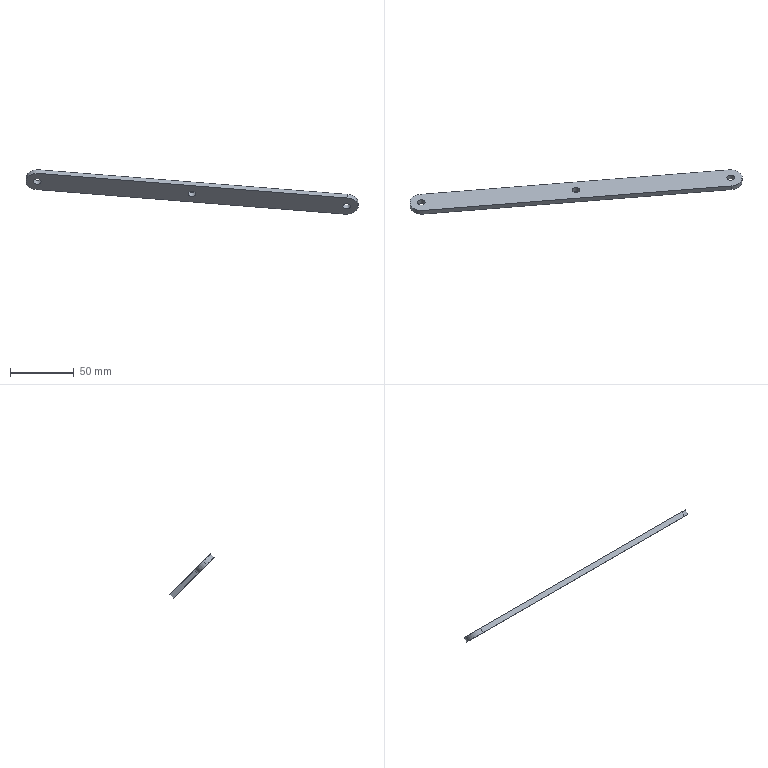Component | SolidWorks | GeneralAssembly-1_TieRod2-1 | 1 solid | 14 faces | box 260.47 x 34.86 x 34.86 mm | volume 18247 mm3 | cylinder 10 | plane 4 | commonest cylinder face diameters 6 x6 18 x4
STEP:
#1=COLOUR_RGB('',0.7922,0.8196,0.9333);
#2=FILL_AREA_STYLE_COLOUR('',#1);
#3=FILL_AREA_STYLE('',(#2));
#4=SURFACE_STYLE_FILL_AREA(#3);
#5=SURFACE_SIDE_STYLE('',(#4));
#6=SURFACE_STYLE_USAGE(.BOTH.,#5);
#7=PRESENTATION_STYLE_ASSIGNMENT((#6));
#8=CARTESIAN_POINT('',(10.928,15.672,-21.042));
#9=VERTEX_POINT('',#8);
#10=CARTESIAN_POINT('',(11.163,15.691,-21.06));
#11=VERTEX_POINT('',#10);
#12=CARTESIAN_POINT('',(11.046,15.682,-21.051));
#13=DIRECTION('',(0.,-0.7071,-0.7071));
#14=DIRECTION('',(0.9937,0.07912,-0.07912));
#15=AXIS2_PLACEMENT_3D('',#12,#13,#14);
#16=CIRCLE('',#15,0.1181);
#17=EDGE_CURVE('',#9,#11,#16,.T.);
#18=ORIENTED_EDGE('',*,*,#17,.F.);
#19=CARTESIAN_POINT('',(10.928,15.561,-21.153));
#20=VERTEX_POINT('',#19);
#21=CARTESIAN_POINT('',(10.928,15.7,-21.014));
#22=DIRECTION('',(0.,-0.7071,-0.7071));
#23=VECTOR('',#22,39.37);
#24=LINE('',#21,#23);
#25=EDGE_CURVE('',#9,#20,#24,.T.);
#26=ORIENTED_EDGE('',*,*,#25,.T.);
#27=CARTESIAN_POINT('',(11.163,15.58,-21.172));
#28=VERTEX_POINT('',#27);
#29=CARTESIAN_POINT('',(11.046,15.57,-21.162));
#30=DIRECTION('',(0.,-0.7071,-0.7071));
#31=DIRECTION('',(0.9937,0.07912,-0.07912));
#32=AXIS2_PLACEMENT_3D('',#29,#30,#31);
#33=CIRCLE('',#32,0.1181);
#34=EDGE_CURVE('',#20,#28,#33,.T.);
#35=ORIENTED_EDGE('',*,*,#34,.T.);
#36=CARTESIAN_POINT('',(11.163,15.719,-21.032));
#37=DIRECTION('',(0.,-0.7071,-0.7071));
#38=VECTOR('',#37,39.37);
#39=LINE('',#36,#38);
#40=EDGE_CURVE('',#11,#28,#39,.T.);
#41=ORIENTED_EDGE('',*,*,#40,.F.);
#42=EDGE_LOOP('',(#18,#26,#35,#41));
#43=FACE_OUTER_BOUND('',#42,.T.);
#44=CARTESIAN_POINT('',(11.046,15.709,-21.023));
#45=DIRECTION('',(0.,-0.7071,-0.7071));
#46=DIRECTION('',(0.9937,0.07912,-0.07912));
#47=AXIS2_PLACEMENT_3D('',#44,#45,#46);
#48=CYLINDRICAL_SURFACE('',#47,0.1181);
#49=ADVANCED_FACE('',(#43),#48,.F.);
#50=CARTESIAN_POINT('',(6.155,15.292,-20.662));
#51=VERTEX_POINT('',#50);
#52=CARTESIAN_POINT('',(6.39,15.311,-20.68));
#53=VERTEX_POINT('',#52);
#54=CARTESIAN_POINT('',(6.273,15.302,-20.671));
#55=DIRECTION('',(0.,-0.7071,-0.7071));
#56=DIRECTION('',(0.9937,0.07912,-0.07912));
#57=AXIS2_PLACEMENT_3D('',#54,#55,#56);
#58=CIRCLE('',#57,0.1181);
#59=EDGE_CURVE('',#51,#53,#58,.T.);
#60=ORIENTED_EDGE('',*,*,#59,.F.);
#61=CARTESIAN_POINT('',(6.155,15.181,-20.773));
#62=VERTEX_POINT('',#61);
#63=CARTESIAN_POINT('',(6.155,15.32,-20.634));
#64=DIRECTION('',(0.,-0.7071,-0.7071));
#65=VECTOR('',#64,39.37);
#66=LINE('',#63,#65);
#67=EDGE_CURVE('',#51,#62,#66,.T.);
#68=ORIENTED_EDGE('',*,*,#67,.T.);
#69=CARTESIAN_POINT('',(6.39,15.2,-20.792));
#70=VERTEX_POINT('',#69);
#71=CARTESIAN_POINT('',(6.273,15.19,-20.782));
#72=DIRECTION('',(0.,-0.7071,-0.7071));
#73=DIRECTION('',(0.9937,0.07912,-0.07912));
#74=AXIS2_PLACEMENT_3D('',#71,#72,#73);
#75=CIRCLE('',#74,0.1181);
#76=EDGE_CURVE('',#62,#70,#75,.T.);
#77=ORIENTED_EDGE('',*,*,#76,.T.);
#78=CARTESIAN_POINT('',(6.39,15.339,-20.652));
#79=DIRECTION('',(0.,-0.7071,-0.7071));
#80=VECTOR('',#79,39.37);
#81=LINE('',#78,#80);
#82=EDGE_CURVE('',#53,#70,#81,.T.);
#83=ORIENTED_EDGE('',*,*,#82,.F.);
#84=EDGE_LOOP('',(#60,#68,#77,#83));
#85=FACE_OUTER_BOUND('',#84,.T.);
#86=CARTESIAN_POINT('',(6.273,15.329,-20.643));
#87=DIRECTION('',(0.,-0.7071,-0.7071));
#88=DIRECTION('',(0.9937,0.07912,-0.07912));
#89=AXIS2_PLACEMENT_3D('',#86,#87,#88);
#90=CYLINDRICAL_SURFACE('',#89,0.1181);
#91=ADVANCED_FACE('',(#85),#90,.F.);
#92=CARTESIAN_POINT('',(1.382,14.912,-20.282));
#93=VERTEX_POINT('',#92);
#94=CARTESIAN_POINT('',(1.617,14.931,-20.3));
#95=VERTEX_POINT('',#94);
#96=CARTESIAN_POINT('',(1.5,14.921,-20.291));
#97=DIRECTION('',(0.,-0.7071,-0.7071));
#98=DIRECTION('',(0.9937,0.07912,-0.07912));
#99=AXIS2_PLACEMENT_3D('',#96,#97,#98);
#100=CIRCLE('',#99,0.1181);
#101=EDGE_CURVE('',#93,#95,#100,.T.);
#102=ORIENTED_EDGE('',*,*,#101,.F.);
#103=CARTESIAN_POINT('',(1.382,14.801,-20.393));
#104=VERTEX_POINT('',#103);
#105=CARTESIAN_POINT('',(1.382,14.94,-20.254));
#106=DIRECTION('',(0.,-0.7071,-0.7071));
#107=VECTOR('',#106,39.37);
#108=LINE('',#105,#107);
#109=EDGE_CURVE('',#93,#104,#108,.T.);
#110=ORIENTED_EDGE('',*,*,#109,.T.);
#111=CARTESIAN_POINT('',(1.617,14.819,-20.412));
#112=VERTEX_POINT('',#111);
#113=CARTESIAN_POINT('',(1.5,14.81,-20.402));
#114=DIRECTION('',(0.,-0.7071,-0.7071));
#115=DIRECTION('',(0.9937,0.07912,-0.07912));
#116=AXIS2_PLACEMENT_3D('',#113,#114,#115);
#117=CIRCLE('',#116,0.1181);
#118=EDGE_CURVE('',#104,#112,#117,.T.);
#119=ORIENTED_EDGE('',*,*,#118,.T.);
#120=CARTESIAN_POINT('',(1.617,14.959,-20.272));
#121=DIRECTION('',(0.,-0.7071,-0.7071));
#122=VECTOR('',#121,39.37);
#123=LINE('',#120,#122);
#124=EDGE_CURVE('',#95,#112,#123,.T.);
#125=ORIENTED_EDGE('',*,*,#124,.F.);
#126=EDGE_LOOP('',(#102,#110,#119,#125));
#127=FACE_OUTER_BOUND('',#126,.T.);
#128=CARTESIAN_POINT('',(1.5,14.949,-20.263));
#129=DIRECTION('',(0.,-0.7071,-0.7071));
#130=DIRECTION('',(0.9937,0.07912,-0.07912));
#131=AXIS2_PLACEMENT_3D('',#128,#129,#130);
#132=CYLINDRICAL_SURFACE('',#131,0.1181);
#133=ADVANCED_FACE('',(#127),#132,.F.);
#134=CARTESIAN_POINT('',(1.46,15.17,-20.54));
#135=VERTEX_POINT('',#134);
#136=CARTESIAN_POINT('',(11.006,15.931,-21.3));
#137=VERTEX_POINT('',#136);
#138=CARTESIAN_POINT('',(1.108,15.142,-20.512));
#139=DIRECTION('',(0.9937,0.07912,-0.07912));
#140=VECTOR('',#139,39.37);
#141=LINE('',#138,#140);
#142=EDGE_CURVE('',#135,#137,#141,.T.);
#143=ORIENTED_EDGE('',*,*,#142,.T.);
#144=CARTESIAN_POINT('',(11.006,15.819,-21.411));
#145=VERTEX_POINT('',#144);
#146=CARTESIAN_POINT('',(11.006,15.819,-21.411));
#147=DIRECTION('',(0.,-0.7071,-0.7071));
#148=VECTOR('',#147,39.37);
#149=LINE('',#146,#148);
#150=EDGE_CURVE('',#137,#145,#149,.T.);
#151=ORIENTED_EDGE('',*,*,#150,.T.);
#152=CARTESIAN_POINT('',(1.46,15.059,-20.651));
#153=VERTEX_POINT('',#152);
#154=CARTESIAN_POINT('',(1.108,15.031,-20.623));
#155=DIRECTION('',(0.9937,0.07912,-0.07912));
#156=VECTOR('',#155,39.37);
#157=LINE('',#154,#156);
#158=EDGE_CURVE('',#153,#145,#157,.T.);
#159=ORIENTED_EDGE('',*,*,#158,.F.);
#160=CARTESIAN_POINT('',(1.46,15.059,-20.651));
#161=DIRECTION('',(-0.,0.7071,0.7071));
#162=VECTOR('',#161,39.37);
#163=LINE('',#160,#162);
#164=EDGE_CURVE('',#153,#135,#163,.T.);
#165=ORIENTED_EDGE('',*,*,#164,.T.);
#166=EDGE_LOOP('',(#143,#151,#159,#165));
#167=FACE_OUTER_BOUND('',#166,.T.);
#168=CARTESIAN_POINT('',(1.108,15.031,-20.623));
#169=DIRECTION('',(0.1119,-0.7027,0.7027));
#170=DIRECTION('',(0.,-0.7071,-0.7071));
#171=AXIS2_PLACEMENT_3D('',#168,#169,#170);
#172=PLANE('',#171);
#173=ADVANCED_FACE('',(#167),#172,.F.);
#174=CARTESIAN_POINT('',(11.085,15.321,-20.913));
#175=VERTEX_POINT('',#174);
#176=CARTESIAN_POINT('',(1.539,14.561,-20.153));
#177=VERTEX_POINT('',#176);
#178=CARTESIAN_POINT('',(1.187,14.533,-20.125));
#179=DIRECTION('',(-0.9937,-0.07912,0.07912));
#180=VECTOR('',#179,39.37);
#181=LINE('',#178,#180);
#182=EDGE_CURVE('',#175,#177,#181,.T.);
#183=ORIENTED_EDGE('',*,*,#182,.F.);
#184=CARTESIAN_POINT('',(11.085,15.433,-20.802));
#185=VERTEX_POINT('',#184);
#186=CARTESIAN_POINT('',(11.085,15.321,-20.913));
#187=DIRECTION('',(-0.,0.7071,0.7071));
#188=VECTOR('',#187,39.37);
#189=LINE('',#186,#188);
#190=EDGE_CURVE('',#175,#185,#189,.T.);
#191=ORIENTED_EDGE('',*,*,#190,.T.);
#192=CARTESIAN_POINT('',(1.539,14.673,-20.042));
#193=VERTEX_POINT('',#192);
#194=CARTESIAN_POINT('',(1.187,14.644,-20.014));
#195=DIRECTION('',(-0.9937,-0.07912,0.07912));
#196=VECTOR('',#195,39.37);
#197=LINE('',#194,#196);
#198=EDGE_CURVE('',#185,#193,#197,.T.);
#199=ORIENTED_EDGE('',*,*,#198,.T.);
#200=CARTESIAN_POINT('',(1.539,14.561,-20.153));
#201=DIRECTION('',(0.,-0.7071,-0.7071));
#202=VECTOR('',#201,39.37);
#203=LINE('',#200,#202);
#204=EDGE_CURVE('',#193,#177,#203,.T.);
#205=ORIENTED_EDGE('',*,*,#204,.T.);
#206=EDGE_LOOP('',(#183,#191,#199,#205));
#207=FACE_OUTER_BOUND('',#206,.T.);
#208=CARTESIAN_POINT('',(1.187,14.533,-20.125));
#209=DIRECTION('',(-0.1119,0.7027,-0.7027));
#210=DIRECTION('',(-0.,0.7071,0.7071));
#211=AXIS2_PLACEMENT_3D('',#208,#209,#210);
#212=PLANE('',#211);
#213=ADVANCED_FACE('',(#207),#212,.F.);
#214=CARTESIAN_POINT('',(11.046,15.57,-21.162));
#215=DIRECTION('',(0.,-0.7071,-0.7071));
#216=DIRECTION('',(0.9937,0.07912,-0.07912));
#217=AXIS2_PLACEMENT_3D('',#214,#215,#216);
#218=CIRCLE('',#217,0.1181);
#219=EDGE_CURVE('',#28,#20,#218,.T.);
#220=ORIENTED_EDGE('',*,*,#219,.F.);
#221=ORIENTED_EDGE('',*,*,#34,.F.);
#222=EDGE_LOOP('',(#220,#221));
#223=FACE_BOUND('',#222,.T.);
#224=CARTESIAN_POINT('',(6.273,15.19,-20.782));
#225=DIRECTION('',(0.,-0.7071,-0.7071));
#226=DIRECTION('',(0.9937,0.07912,-0.07912));
#227=AXIS2_PLACEMENT_3D('',#224,#225,#226);
#228=CIRCLE('',#227,0.1181);
#229=EDGE_CURVE('',#70,#62,#228,.T.);
#230=ORIENTED_EDGE('',*,*,#229,.F.);
#231=ORIENTED_EDGE('',*,*,#76,.F.);
#232=EDGE_LOOP('',(#230,#231));
#233=FACE_BOUND('',#232,.T.);
#234=CARTESIAN_POINT('',(1.5,14.81,-20.402));
#235=DIRECTION('',(0.,-0.7071,-0.7071));
#236=DIRECTION('',(0.9937,0.07912,-0.07912));
#237=AXIS2_PLACEMENT_3D('',#234,#235,#236);
#238=CIRCLE('',#237,0.1181);
#239=EDGE_CURVE('',#112,#104,#238,.T.);
#240=ORIENTED_EDGE('',*,*,#239,.F.);
#241=ORIENTED_EDGE('',*,*,#118,.F.);
#242=EDGE_LOOP('',(#240,#241));
#243=FACE_BOUND('',#242,.T.);
#244=ORIENTED_EDGE('',*,*,#158,.T.);
#245=CARTESIAN_POINT('',(11.398,15.598,-21.19));
#246=VERTEX_POINT('',#245);
#247=CARTESIAN_POINT('',(11.046,15.57,-21.162));
#248=DIRECTION('',(0.,-0.7071,-0.7071));
#249=DIRECTION('',(0.9937,0.07912,-0.07912));
#250=AXIS2_PLACEMENT_3D('',#247,#248,#249);
#251=CIRCLE('',#250,0.3543);
#252=EDGE_CURVE('',#145,#246,#251,.T.);
#253=ORIENTED_EDGE('',*,*,#252,.T.);
#254=CARTESIAN_POINT('',(11.046,15.57,-21.162));
#255=DIRECTION('',(0.,-0.7071,-0.7071));
#256=DIRECTION('',(0.9937,0.07912,-0.07912));
#257=AXIS2_PLACEMENT_3D('',#254,#255,#256);
#258=CIRCLE('',#257,0.3543);
#259=EDGE_CURVE('',#246,#175,#258,.T.);
#260=ORIENTED_EDGE('',*,*,#259,.T.);
#261=ORIENTED_EDGE('',*,*,#182,.T.);
#262=CARTESIAN_POINT('',(1.148,14.782,-20.374));
#263=VERTEX_POINT('',#262);
#264=CARTESIAN_POINT('',(1.5,14.81,-20.402));
#265=DIRECTION('',(0.,-0.7071,-0.7071));
#266=DIRECTION('',(0.9937,0.07912,-0.07912));
#267=AXIS2_PLACEMENT_3D('',#264,#265,#266);
#268=CIRCLE('',#267,0.3543);
#269=EDGE_CURVE('',#177,#263,#268,.T.);
#270=ORIENTED_EDGE('',*,*,#269,.T.);
#271=CARTESIAN_POINT('',(1.5,14.81,-20.402));
#272=DIRECTION('',(0.,-0.7071,-0.7071));
#273=DIRECTION('',(0.9937,0.07912,-0.07912));
#274=AXIS2_PLACEMENT_3D('',#271,#272,#273);
#275=CIRCLE('',#274,0.3543);
#276=EDGE_CURVE('',#263,#153,#275,.T.);
#277=ORIENTED_EDGE('',*,*,#276,.T.);
#278=EDGE_LOOP('',(#244,#253,#260,#261,#270,#277));
#279=FACE_OUTER_BOUND('',#278,.T.);
#280=CARTESIAN_POINT('',(3.616,15.166,-20.758));
#281=DIRECTION('',(0.,-0.7071,-0.7071));
#282=DIRECTION('',(0.9937,0.07912,-0.07912));
#283=AXIS2_PLACEMENT_3D('',#280,#281,#282);
#284=PLANE('',#283);
#285=ADVANCED_FACE('',(#223,#233,#243,#279),#284,.T.);
#286=CARTESIAN_POINT('',(11.046,15.682,-21.051));
#287=DIRECTION('',(0.,-0.7071,-0.7071));
#288=DIRECTION('',(0.9937,0.07912,-0.07912));
#289=AXIS2_PLACEMENT_3D('',#286,#287,#288);
#290=CIRCLE('',#289,0.1181);
#291=EDGE_CURVE('',#11,#9,#290,.T.);
#292=ORIENTED_EDGE('',*,*,#291,.T.);
#293=ORIENTED_EDGE('',*,*,#17,.T.);
#294=EDGE_LOOP('',(#292,#293));
#295=FACE_BOUND('',#294,.T.);
#296=CARTESIAN_POINT('',(6.273,15.302,-20.671));
#297=DIRECTION('',(0.,-0.7071,-0.7071));
#298=DIRECTION('',(0.9937,0.07912,-0.07912));
#299=AXIS2_PLACEMENT_3D('',#296,#297,#298);
#300=CIRCLE('',#299,0.1181);
#301=EDGE_CURVE('',#53,#51,#300,.T.);
#302=ORIENTED_EDGE('',*,*,#301,.T.);
#303=ORIENTED_EDGE('',*,*,#59,.T.);
#304=EDGE_LOOP('',(#302,#303));
#305=FACE_BOUND('',#304,.T.);
#306=CARTESIAN_POINT('',(1.5,14.921,-20.291));
#307=DIRECTION('',(0.,-0.7071,-0.7071));
#308=DIRECTION('',(0.9937,0.07912,-0.07912));
#309=AXIS2_PLACEMENT_3D('',#306,#307,#308);
#310=CIRCLE('',#309,0.1181);
#311=EDGE_CURVE('',#95,#93,#310,.T.);
#312=ORIENTED_EDGE('',*,*,#311,.T.);
#313=ORIENTED_EDGE('',*,*,#101,.T.);
#314=EDGE_LOOP('',(#312,#313));
#315=FACE_BOUND('',#314,.T.);
#316=CARTESIAN_POINT('',(11.398,15.71,-21.079));
#317=VERTEX_POINT('',#316);
#318=CARTESIAN_POINT('',(11.046,15.682,-21.051));
#319=DIRECTION('',(-0.,0.7071,0.7071));
#320=DIRECTION('',(0.9937,0.07912,-0.07912));
#321=AXIS2_PLACEMENT_3D('',#318,#319,#320);
#322=CIRCLE('',#321,0.3543);
#323=EDGE_CURVE('',#185,#317,#322,.T.);
#324=ORIENTED_EDGE('',*,*,#323,.T.);
#325=CARTESIAN_POINT('',(11.046,15.682,-21.051));
#326=DIRECTION('',(-0.,0.7071,0.7071));
#327=DIRECTION('',(0.9937,0.07912,-0.07912));
#328=AXIS2_PLACEMENT_3D('',#325,#326,#327);
#329=CIRCLE('',#328,0.3543);
#330=EDGE_CURVE('',#317,#137,#329,.T.);
#331=ORIENTED_EDGE('',*,*,#330,.T.);
#332=ORIENTED_EDGE('',*,*,#142,.F.);
#333=CARTESIAN_POINT('',(1.148,14.893,-20.263));
#334=VERTEX_POINT('',#333);
#335=CARTESIAN_POINT('',(1.5,14.921,-20.291));
#336=DIRECTION('',(-0.,0.7071,0.7071));
#337=DIRECTION('',(0.9937,0.07912,-0.07912));
#338=AXIS2_PLACEMENT_3D('',#335,#336,#337);
#339=CIRCLE('',#338,0.3543);
#340=EDGE_CURVE('',#135,#334,#339,.T.);
#341=ORIENTED_EDGE('',*,*,#340,.T.);
#342=CARTESIAN_POINT('',(1.5,14.921,-20.291));
#343=DIRECTION('',(-0.,0.7071,0.7071));
#344=DIRECTION('',(0.9937,0.07912,-0.07912));
#345=AXIS2_PLACEMENT_3D('',#342,#343,#344);
#346=CIRCLE('',#345,0.3543);
#347=EDGE_CURVE('',#334,#193,#346,.T.);
#348=ORIENTED_EDGE('',*,*,#347,.T.);
#349=ORIENTED_EDGE('',*,*,#198,.F.);
#350=EDGE_LOOP('',(#324,#331,#332,#341,#348,#349));
#351=FACE_OUTER_BOUND('',#350,.T.);
#352=CARTESIAN_POINT('',(3.616,15.277,-20.647));
#353=DIRECTION('',(0.,-0.7071,-0.7071));
#354=DIRECTION('',(0.9937,0.07912,-0.07912));
#355=AXIS2_PLACEMENT_3D('',#352,#353,#354);
#356=PLANE('',#355);
#357=ADVANCED_FACE('',(#295,#305,#315,#351),#356,.F.);
#358=ORIENTED_EDGE('',*,*,#190,.F.);
#359=ORIENTED_EDGE('',*,*,#259,.F.);
#360=CARTESIAN_POINT('',(11.398,15.598,-21.19));
#361=DIRECTION('',(0.,-0.7071,-0.7071));
#362=VECTOR('',#361,39.37);
#363=LINE('',#360,#362);
#364=EDGE_CURVE('',#317,#246,#363,.T.);
#365=ORIENTED_EDGE('',*,*,#364,.F.);
#366=ORIENTED_EDGE('',*,*,#323,.F.);
#367=EDGE_LOOP('',(#358,#359,#365,#366));
#368=FACE_OUTER_BOUND('',#367,.T.);
#369=CARTESIAN_POINT('',(11.046,15.57,-21.162));
#370=DIRECTION('',(-0.,0.7071,0.7071));
#371=DIRECTION('',(-0.9937,-0.07912,0.07912));
#372=AXIS2_PLACEMENT_3D('',#369,#370,#371);
#373=CYLINDRICAL_SURFACE('',#372,0.3543);
#374=ADVANCED_FACE('',(#368),#373,.T.);
#375=ORIENTED_EDGE('',*,*,#252,.F.);
#376=ORIENTED_EDGE('',*,*,#150,.F.);
#377=ORIENTED_EDGE('',*,*,#330,.F.);
#378=ORIENTED_EDGE('',*,*,#364,.T.);
#379=EDGE_LOOP('',(#375,#376,#377,#378));
#380=FACE_OUTER_BOUND('',#379,.T.);
#381=CARTESIAN_POINT('',(11.046,15.57,-21.162));
#382=DIRECTION('',(-0.,0.7071,0.7071));
#383=DIRECTION('',(-0.9937,-0.07912,0.07912));
#384=AXIS2_PLACEMENT_3D('',#381,#382,#383);
#385=CYLINDRICAL_SURFACE('',#384,0.3543);
#386=ADVANCED_FACE('',(#380),#385,.T.);
#387=CARTESIAN_POINT('',(1.148,14.782,-20.374));
#388=DIRECTION('',(-0.,0.7071,0.7071));
#389=VECTOR('',#388,39.37);
#390=LINE('',#387,#389);
#391=EDGE_CURVE('',#263,#334,#390,.T.);
#392=ORIENTED_EDGE('',*,*,#391,.F.);
#393=ORIENTED_EDGE('',*,*,#269,.F.);
#394=ORIENTED_EDGE('',*,*,#204,.F.);
#395=ORIENTED_EDGE('',*,*,#347,.F.);
#396=EDGE_LOOP('',(#392,#393,#394,#395));
#397=FACE_OUTER_BOUND('',#396,.T.);
#398=CARTESIAN_POINT('',(1.5,14.81,-20.402));
#399=DIRECTION('',(-0.,0.7071,0.7071));
#400=DIRECTION('',(-0.9937,-0.07912,0.07912));
#401=AXIS2_PLACEMENT_3D('',#398,#399,#400);
#402=CYLINDRICAL_SURFACE('',#401,0.3543);
#403=ADVANCED_FACE('',(#397),#402,.T.);
#404=ORIENTED_EDGE('',*,*,#276,.F.);
#405=ORIENTED_EDGE('',*,*,#391,.T.);
#406=ORIENTED_EDGE('',*,*,#340,.F.);
#407=ORIENTED_EDGE('',*,*,#164,.F.);
#408=EDGE_LOOP('',(#404,#405,#406,#407));
#409=FACE_OUTER_BOUND('',#408,.T.);
#410=CARTESIAN_POINT('',(1.5,14.81,-20.402));
#411=DIRECTION('',(-0.,0.7071,0.7071));
#412=DIRECTION('',(-0.9937,-0.07912,0.07912));
#413=AXIS2_PLACEMENT_3D('',#410,#411,#412);
#414=CYLINDRICAL_SURFACE('',#413,0.3543);
#415=ADVANCED_FACE('',(#409),#414,.T.);
#416=ORIENTED_EDGE('',*,*,#109,.F.);
#417=ORIENTED_EDGE('',*,*,#311,.F.);
#418=ORIENTED_EDGE('',*,*,#124,.T.);
#419=ORIENTED_EDGE('',*,*,#239,.T.);
#420=EDGE_LOOP('',(#416,#417,#418,#419));
#421=FACE_OUTER_BOUND('',#420,.T.);
#422=CARTESIAN_POINT('',(1.5,14.949,-20.263));
#423=DIRECTION('',(0.,-0.7071,-0.7071));
#424=DIRECTION('',(0.9937,0.07912,-0.07912));
#425=AXIS2_PLACEMENT_3D('',#422,#423,#424);
#426=CYLINDRICAL_SURFACE('',#425,0.1181);
#427=ADVANCED_FACE('',(#421),#426,.F.);
#428=ORIENTED_EDGE('',*,*,#67,.F.);
#429=ORIENTED_EDGE('',*,*,#301,.F.);
#430=ORIENTED_EDGE('',*,*,#82,.T.);
#431=ORIENTED_EDGE('',*,*,#229,.T.);
#432=EDGE_LOOP('',(#428,#429,#430,#431));
#433=FACE_OUTER_BOUND('',#432,.T.);
#434=CARTESIAN_POINT('',(6.273,15.329,-20.643));
#435=DIRECTION('',(0.,-0.7071,-0.7071));
#436=DIRECTION('',(0.9937,0.07912,-0.07912));
#437=AXIS2_PLACEMENT_3D('',#434,#435,#436);
#438=CYLINDRICAL_SURFACE('',#437,0.1181);
#439=ADVANCED_FACE('',(#433),#438,.F.);
#440=ORIENTED_EDGE('',*,*,#25,.F.);
#441=ORIENTED_EDGE('',*,*,#291,.F.);
#442=ORIENTED_EDGE('',*,*,#40,.T.);
#443=ORIENTED_EDGE('',*,*,#219,.T.);
#444=EDGE_LOOP('',(#440,#441,#442,#443));
#445=FACE_OUTER_BOUND('',#444,.T.);
#446=CARTESIAN_POINT('',(11.046,15.709,-21.023));
#447=DIRECTION('',(0.,-0.7071,-0.7071));
#448=DIRECTION('',(0.9937,0.07912,-0.07912));
#449=AXIS2_PLACEMENT_3D('',#446,#447,#448);
#450=CYLINDRICAL_SURFACE('',#449,0.1181);
#451=ADVANCED_FACE('',(#445),#450,.F.);
#452=CLOSED_SHELL('',(#49,#91,#133,#173,#213,#285,#357,#374,#386,#403,#415,#427,#439,#451));
#453=MANIFOLD_SOLID_BREP('',#452);
#454=STYLED_ITEM('',(#7),#453);
#455=(LENGTH_UNIT()NAMED_UNIT(*)SI_UNIT($,.METRE.));
#456=LENGTH_MEASURE_WITH_UNIT(LENGTH_MEASURE(0.0254),#455);
#457=DIMENSIONAL_EXPONENTS(1.,0.,0.,0.,0.,0.,0.);
#458=(CONVERSION_BASED_UNIT('',#456)LENGTH_UNIT()NAMED_UNIT(#457));
#459=UNCERTAINTY_MEASURE_WITH_UNIT(LENGTH_MEASURE(0.00001),#458,'','');
#460=(NAMED_UNIT(*)PLANE_ANGLE_UNIT()SI_UNIT($,.RADIAN.));
#461=(NAMED_UNIT(*)SI_UNIT($,.STERADIAN.)SOLID_ANGLE_UNIT());
#462=(GEOMETRIC_REPRESENTATION_CONTEXT(3)GLOBAL_UNCERTAINTY_ASSIGNED_CONTEXT((#459))GLOBAL_UNIT_ASSIGNED_CONTEXT((#458,#460,#461))REPRESENTATION_CONTEXT('',''));
#463=MECHANICAL_DESIGN_GEOMETRIC_PRESENTATION_REPRESENTATION('',(#454),#462);
#464=CARTESIAN_POINT('',(0.,0.,0.));
#465=DIRECTION('',(0.,0.,1.));
#466=DIRECTION('',(1.,0.,0.));
#467=AXIS2_PLACEMENT_3D('',#464,#465,#466);
#468=(LENGTH_UNIT()NAMED_UNIT(*)SI_UNIT($,.METRE.));
#469=LENGTH_MEASURE_WITH_UNIT(LENGTH_MEASURE(0.0254),#468);
#470=DIMENSIONAL_EXPONENTS(1.,0.,0.,0.,0.,0.,0.);
#471=(CONVERSION_BASED_UNIT('',#469)LENGTH_UNIT()NAMED_UNIT(#470));
#472=UNCERTAINTY_MEASURE_WITH_UNIT(LENGTH_MEASURE(0.00001),#471,'','');
#473=(NAMED_UNIT(*)PLANE_ANGLE_UNIT()SI_UNIT($,.RADIAN.));
#474=(NAMED_UNIT(*)SI_UNIT($,.STERADIAN.)SOLID_ANGLE_UNIT());
#475=(GEOMETRIC_REPRESENTATION_CONTEXT(3)GLOBAL_UNCERTAINTY_ASSIGNED_CONTEXT((#472))GLOBAL_UNIT_ASSIGNED_CONTEXT((#471,#473,#474))REPRESENTATION_CONTEXT('',''));
#476=ADVANCED_BREP_SHAPE_REPRESENTATION('',(#453,#467),#475);
#477=PRESENTATION_LAYER_ASSIGNMENT('','',(#454));